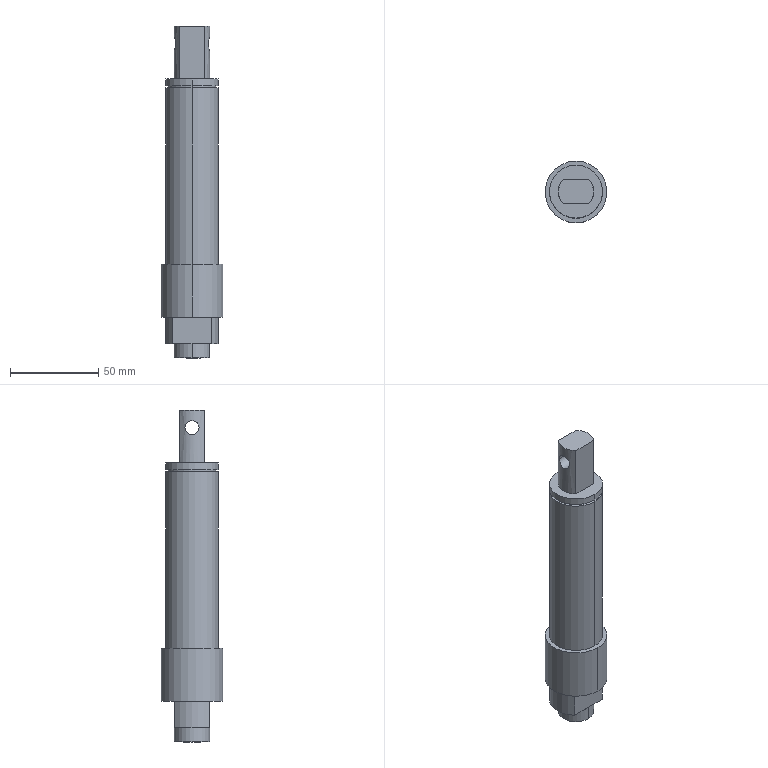Component | SolidWorks | -DrivenPulleyShaft-1 | 1 solid | 33 faces | box 35 x 35 x 188 mm | volume 119550 mm3 | cylinder 18 | plane 13 | cone 2 | commonest cylinder face diameters 30 x6 20 x4 8 x2 6.8 x2 35 x2 27 x2
build123d program:
from build123d import *

# Parameters (mm, degrees)
SKETCH2_W             = 5.308
SKETCH2_H             = 29.965
SKETCH2_W_2           = 6.945
SKETCH2_H_2           = 31.552
CUT_EXTRUDE1_DEPTH    = 15
M8_TAPPED_HOLE1_D     = 6.8
M8_TAPPED_HOLE1_DEPTH = 22.25
M8_TAPPED_HOLE1_TIP   = 2.043
SKETCH5_W             = 20.068
SKETCH5_H             = 42.894
SKETCH5_W_2           = 13.481
SKETCH5_H_2           = 39.37
CUT_EXTRUDE3_DEPTH    = 30
M8_TAPPED_HOLE2_D     = 8


with BuildPart() as part:
    # Sketch1 → Revolve1 (revolve)
    with BuildSketch(Plane(origin=(0, 0, 0), x_dir=(1, 0, 0), z_dir=(0, 1, 0)), mode=Mode.PRIVATE) as revolve1_sk:
        Polygon((0, 0), (0, 10), (30, 10), (30, 15), (33.8, 15), (33.8, 13.5), (35, 13.5), (35, 15), (135, 15), (135, 17.5), (165, 17.5), (165, 15), (180, 15), (180, 10), (188, 10), (188, 0), align=None)
    revolve(revolve1_sk.sketch.rotate(Axis((-511.379, 0, 0), (1, 0, 0)), 180), axis=Axis((-511.379, 0, 0), (1, 0, 0)))

    # Sketch2 → Cut-Extrude1 (cut)
    with BuildSketch(Plane(origin=(180, 0, 0), x_dir=(0, 0, -1), z_dir=(1, 0, 0))):
        with Locations((-12.654, -0.3473)):
            Rectangle(SKETCH2_W, SKETCH2_H)
        with Locations((13.473, -1.141)):
            Rectangle(SKETCH2_W_2, SKETCH2_H_2)
    extrude(amount=-CUT_EXTRUDE1_DEPTH, mode=Mode.SUBTRACT)

    # M8 Tapped Hole1
    with Locations(Plane(origin=(188, 0, 0), x_dir=(0, 0, -1), z_dir=(1, 0, 0))):
        with Locations((0, 0)):
            Hole(M8_TAPPED_HOLE1_D / 2, depth=M8_TAPPED_HOLE1_DEPTH)
            with Locations((0, 0, -(M8_TAPPED_HOLE1_DEPTH + M8_TAPPED_HOLE1_TIP / 2))):  # 118° drill point
                Cone(0, M8_TAPPED_HOLE1_D / 2, M8_TAPPED_HOLE1_TIP, mode=Mode.SUBTRACT)

    # Sketch5 → Cut-Extrude3 (cut)
    with BuildSketch(Plane.ZY):
        with Locations((-17.034, -1.358)):
            Rectangle(SKETCH5_W, SKETCH5_H)
        with Locations((13.74, -4.805)):
            Rectangle(SKETCH5_W_2, SKETCH5_H_2)
    extrude(amount=-CUT_EXTRUDE3_DEPTH, mode=Mode.SUBTRACT)

    # M8 Tapped Hole2 (through all)
    with Locations(Plane(origin=(0, -10, 0), x_dir=(-1, 0, 0), z_dir=(0, -1, 0))):
        with Locations((-10, 0)):
            Hole(M8_TAPPED_HOLE2_D / 2)


solid = part.part

# Placed as in the assembly
solid = solid.moved(Location((-130, 1094.5, 170), (90, 0, -90)))
STEP:
#1=COLOUR_RGB('',0.7922,0.8196,0.9333);
#2=FILL_AREA_STYLE_COLOUR('',#1);
#3=FILL_AREA_STYLE('',(#2));
#4=SURFACE_STYLE_FILL_AREA(#3);
#5=SURFACE_SIDE_STYLE('',(#4));
#6=SURFACE_STYLE_USAGE(.BOTH.,#5);
#7=PRESENTATION_STYLE_ASSIGNMENT((#6));
#8=CARTESIAN_POINT('',(-5.479,43.248,6.299));
#9=VERTEX_POINT('',#8);
#10=CARTESIAN_POINT('',(-5.479,42.933,6.299));
#11=VERTEX_POINT('',#10);
#12=CARTESIAN_POINT('',(-5.479,43.248,6.299));
#13=CARTESIAN_POINT('',(-5.479,43.248,6.31));
#14=CARTESIAN_POINT('',(-5.479,43.247,6.32));
#15=CARTESIAN_POINT('',(-5.481,43.243,6.34));
#16=CARTESIAN_POINT('',(-5.482,43.24,6.35));
#17=CARTESIAN_POINT('',(-5.486,43.232,6.369));
#18=CARTESIAN_POINT('',(-5.487,43.227,6.378));
#19=CARTESIAN_POINT('',(-5.491,43.216,6.395));
#20=CARTESIAN_POINT('',(-5.494,43.209,6.403));
#21=CARTESIAN_POINT('',(-5.498,43.195,6.418));
#22=CARTESIAN_POINT('',(-5.5,43.187,6.424));
#23=CARTESIAN_POINT('',(-5.504,43.17,6.436));
#24=CARTESIAN_POINT('',(-5.506,43.161,6.441));
#25=CARTESIAN_POINT('',(-5.509,43.142,6.449));
#26=CARTESIAN_POINT('',(-5.51,43.132,6.452));
#27=CARTESIAN_POINT('',(-5.511,43.112,6.456));
#28=CARTESIAN_POINT('',(-5.512,43.101,6.457));
#29=CARTESIAN_POINT('',(-5.512,43.08,6.457));
#30=CARTESIAN_POINT('',(-5.511,43.07,6.456));
#31=CARTESIAN_POINT('',(-5.51,43.049,6.452));
#32=CARTESIAN_POINT('',(-5.509,43.039,6.449));
#33=CARTESIAN_POINT('',(-5.506,43.021,6.441));
#34=CARTESIAN_POINT('',(-5.504,43.011,6.436));
#35=CARTESIAN_POINT('',(-5.5,42.994,6.424));
#36=CARTESIAN_POINT('',(-5.498,42.986,6.418));
#37=CARTESIAN_POINT('',(-5.494,42.972,6.403));
#38=CARTESIAN_POINT('',(-5.491,42.965,6.395));
#39=CARTESIAN_POINT('',(-5.487,42.954,6.379));
#40=CARTESIAN_POINT('',(-5.486,42.949,6.37));
#41=CARTESIAN_POINT('',(-5.482,42.941,6.35));
#42=CARTESIAN_POINT('',(-5.481,42.938,6.34));
#43=CARTESIAN_POINT('',(-5.479,42.934,6.32));
#44=CARTESIAN_POINT('',(-5.479,42.933,6.31));
#45=CARTESIAN_POINT('',(-5.479,42.933,6.299));
#46=B_SPLINE_CURVE_WITH_KNOTS('',3,(#12,#13,#14,#15,#16,#17,#18,#19,#20,#21,#22,#23,#24,#25,#26,#27,#28,#29,#30,#31,#32,#33,#34,#35,#36,#37,#38,#39,#40,#41,#42,#43,#44,#45),.UNSPECIFIED.,.F.,.F.,(4,2,2,2,2,2,2,2,2,2,2,2,2,2,2,2,4),(0.01264,0.01343,0.01422,0.01501,0.0158,0.01658,0.01737,0.01816,0.01895,0.01974,0.02053,0.02132,0.02211,0.0229,0.02369,0.02448,0.02527),.UNSPECIFIED.);
#47=EDGE_CURVE('',#9,#11,#46,.T.);
#48=ORIENTED_EDGE('',*,*,#47,.F.);
#49=CARTESIAN_POINT('',(-4.757,43.248,6.299));
#50=VERTEX_POINT('',#49);
#51=CARTESIAN_POINT('',(-4.724,43.248,6.299));
#52=DIRECTION('',(1.,0.,-0.));
#53=VECTOR('',#52,39.37);
#54=LINE('',#51,#53);
#55=EDGE_CURVE('',#9,#50,#54,.T.);
#56=ORIENTED_EDGE('',*,*,#55,.T.);
#57=CARTESIAN_POINT('',(-4.757,42.933,6.299));
#58=VERTEX_POINT('',#57);
#59=CARTESIAN_POINT('',(-4.757,42.933,6.299));
#60=CARTESIAN_POINT('',(-4.757,42.933,6.31));
#61=CARTESIAN_POINT('',(-4.757,42.934,6.32));
#62=CARTESIAN_POINT('',(-4.755,42.938,6.34));
#63=CARTESIAN_POINT('',(-4.754,42.941,6.35));
#64=CARTESIAN_POINT('',(-4.751,42.949,6.369));
#65=CARTESIAN_POINT('',(-4.749,42.954,6.378));
#66=CARTESIAN_POINT('',(-4.745,42.965,6.395));
#67=CARTESIAN_POINT('',(-4.743,42.972,6.403));
#68=CARTESIAN_POINT('',(-4.738,42.986,6.418));
#69=CARTESIAN_POINT('',(-4.736,42.994,6.424));
#70=CARTESIAN_POINT('',(-4.732,43.011,6.436));
#71=CARTESIAN_POINT('',(-4.731,43.02,6.441));
#72=CARTESIAN_POINT('',(-4.728,43.039,6.448));
#73=CARTESIAN_POINT('',(-4.726,43.049,6.452));
#74=CARTESIAN_POINT('',(-4.725,43.07,6.456));
#75=CARTESIAN_POINT('',(-4.724,43.08,6.457));
#76=CARTESIAN_POINT('',(-4.724,43.101,6.457));
#77=CARTESIAN_POINT('',(-4.725,43.111,6.456));
#78=CARTESIAN_POINT('',(-4.726,43.132,6.452));
#79=CARTESIAN_POINT('',(-4.728,43.142,6.449));
#80=CARTESIAN_POINT('',(-4.731,43.161,6.441));
#81=CARTESIAN_POINT('',(-4.732,43.17,6.436));
#82=CARTESIAN_POINT('',(-4.736,43.187,6.424));
#83=CARTESIAN_POINT('',(-4.738,43.195,6.418));
#84=CARTESIAN_POINT('',(-4.743,43.209,6.403));
#85=CARTESIAN_POINT('',(-4.745,43.216,6.395));
#86=CARTESIAN_POINT('',(-4.749,43.227,6.378));
#87=CARTESIAN_POINT('',(-4.751,43.232,6.369));
#88=CARTESIAN_POINT('',(-4.754,43.24,6.35));
#89=CARTESIAN_POINT('',(-4.755,43.243,6.34));
#90=CARTESIAN_POINT('',(-4.757,43.247,6.32));
#91=CARTESIAN_POINT('',(-4.757,43.248,6.31));
#92=CARTESIAN_POINT('',(-4.757,43.248,6.299));
#93=B_SPLINE_CURVE_WITH_KNOTS('',3,(#59,#60,#61,#62,#63,#64,#65,#66,#67,#68,#69,#70,#71,#72,#73,#74,#75,#76,#77,#78,#79,#80,#81,#82,#83,#84,#85,#86,#87,#88,#89,#90,#91,#92),.UNSPECIFIED.,.F.,.F.,(4,2,2,2,2,2,2,2,2,2,2,2,2,2,2,2,4),(0.,0.0007899,0.00158,0.00237,0.00316,0.00395,0.00474,0.00553,0.006319,0.007109,0.007899,0.008689,0.009479,0.01027,0.01106,0.01185,0.01264),.UNSPECIFIED.);
#94=EDGE_CURVE('',#58,#50,#93,.T.);
#95=ORIENTED_EDGE('',*,*,#94,.F.);
#96=CARTESIAN_POINT('',(-4.724,42.933,6.299));
#97=DIRECTION('',(1.,0.,-0.));
#98=VECTOR('',#97,39.37);
#99=LINE('',#96,#98);
#100=EDGE_CURVE('',#11,#58,#99,.T.);
#101=ORIENTED_EDGE('',*,*,#100,.F.);
#102=EDGE_LOOP('',(#48,#56,#95,#101));
#103=FACE_OUTER_BOUND('',#102,.T.);
#104=CARTESIAN_POINT('',(-4.724,43.091,6.299));
#105=DIRECTION('',(1.,0.,-0.));
#106=DIRECTION('',(0.,-1.,0.));
#107=AXIS2_PLACEMENT_3D('',#104,#105,#106);
#108=CYLINDRICAL_SURFACE('',#107,0.1575);
#109=ADVANCED_FACE('',(#103),#108,.F.);
#110=CARTESIAN_POINT('',(-5.118,43.224,0.1673));
#111=VERTEX_POINT('',#110);
#112=CARTESIAN_POINT('',(-5.118,42.957,0.1673));
#113=VERTEX_POINT('',#112);
#114=CARTESIAN_POINT('',(-5.118,43.091,0.1673));
#115=DIRECTION('',(-0.,-0.,-1.));
#116=DIRECTION('',(0.,-1.,0.));
#117=AXIS2_PLACEMENT_3D('',#114,#115,#116);
#118=CIRCLE('',#117,0.1339);
#119=EDGE_CURVE('',#111,#113,#118,.T.);
#120=ORIENTED_EDGE('',*,*,#119,.F.);
#121=CARTESIAN_POINT('',(-5.118,43.224,-0.7087));
#122=VERTEX_POINT('',#121);
#123=CARTESIAN_POINT('',(-5.118,43.224,-0.7087));
#124=DIRECTION('',(-0.,-0.,-1.));
#125=VECTOR('',#124,39.37);
#126=LINE('',#123,#125);
#127=EDGE_CURVE('',#111,#122,#126,.T.);
#128=ORIENTED_EDGE('',*,*,#127,.T.);
#129=CARTESIAN_POINT('',(-5.118,42.957,-0.7087));
#130=VERTEX_POINT('',#129);
#131=CARTESIAN_POINT('',(-5.118,43.091,-0.7087));
#132=DIRECTION('',(-0.,-0.,-1.));
#133=DIRECTION('',(0.,-1.,0.));
#134=AXIS2_PLACEMENT_3D('',#131,#132,#133);
#135=CIRCLE('',#134,0.1339);
#136=EDGE_CURVE('',#122,#130,#135,.T.);
#137=ORIENTED_EDGE('',*,*,#136,.T.);
#138=CARTESIAN_POINT('',(-5.118,42.957,-0.7087));
#139=DIRECTION('',(-0.,-0.,-1.));
#140=VECTOR('',#139,39.37);
#141=LINE('',#138,#140);
#142=EDGE_CURVE('',#113,#130,#141,.T.);
#143=ORIENTED_EDGE('',*,*,#142,.F.);
#144=EDGE_LOOP('',(#120,#128,#137,#143));
#145=FACE_OUTER_BOUND('',#144,.T.);
#146=CARTESIAN_POINT('',(-5.118,43.091,-0.7087));
#147=DIRECTION('',(-0.,-0.,-1.));
#148=DIRECTION('',(0.,-1.,0.));
#149=AXIS2_PLACEMENT_3D('',#146,#147,#148);
#150=CYLINDRICAL_SURFACE('',#149,0.1339);
#151=ADVANCED_FACE('',(#145),#150,.F.);
#152=CARTESIAN_POINT('',(-5.118,43.091,0.2478));
#153=VERTEX_POINT('',#152);
#154=CARTESIAN_POINT('',(-5.118,42.957,0.1673));
#155=DIRECTION('',(0.,-0.8572,-0.515));
#156=VECTOR('',#155,39.37);
#157=LINE('',#154,#156);
#158=EDGE_CURVE('',#153,#113,#157,.T.);
#159=ORIENTED_EDGE('',*,*,#158,.F.);
#160=CARTESIAN_POINT('',(-5.118,43.224,0.1673));
#161=DIRECTION('',(-0.,0.8572,-0.515));
#162=VECTOR('',#161,39.37);
#163=LINE('',#160,#162);
#164=EDGE_CURVE('',#153,#111,#163,.T.);
#165=ORIENTED_EDGE('',*,*,#164,.T.);
#166=ORIENTED_EDGE('',*,*,#119,.T.);
#167=EDGE_LOOP('',(#159,#165,#166));
#168=FACE_OUTER_BOUND('',#167,.T.);
#169=CARTESIAN_POINT('',(-5.118,43.091,0.1673));
#170=DIRECTION('',(-0.,-0.,-1.));
#171=DIRECTION('',(0.,-1.,0.));
#172=AXIS2_PLACEMENT_3D('',#169,#170,#171);
#173=CONICAL_SURFACE('',#172,0.1339,1.03);
#174=ADVANCED_FACE('',(#168),#173,.F.);
#175=CARTESIAN_POINT('',(-5.118,43.484,-0.7087));
#176=VERTEX_POINT('',#175);
#177=CARTESIAN_POINT('',(-5.118,42.697,-0.7087));
#178=VERTEX_POINT('',#177);
#179=CARTESIAN_POINT('',(-5.118,43.091,-0.7087));
#180=DIRECTION('',(0.,0.,1.));
#181=DIRECTION('',(-0.,1.,0.));
#182=AXIS2_PLACEMENT_3D('',#179,#180,#181);
#183=CIRCLE('',#182,0.3937);
#184=EDGE_CURVE('',#176,#178,#183,.T.);
#185=ORIENTED_EDGE('',*,*,#184,.T.);
#186=CARTESIAN_POINT('',(-5.118,42.697,-0.3937));
#187=VERTEX_POINT('',#186);
#188=CARTESIAN_POINT('',(-5.118,42.697,26.826));
#189=DIRECTION('',(0.,0.,1.));
#190=VECTOR('',#189,39.37);
#191=LINE('',#188,#190);
#192=EDGE_CURVE('',#178,#187,#191,.T.);
#193=ORIENTED_EDGE('',*,*,#192,.T.);
#194=CARTESIAN_POINT('',(-5.118,43.484,-0.3937));
#195=VERTEX_POINT('',#194);
#196=CARTESIAN_POINT('',(-5.118,43.091,-0.3937));
#197=DIRECTION('',(0.,0.,1.));
#198=DIRECTION('',(-0.,1.,0.));
#199=AXIS2_PLACEMENT_3D('',#196,#197,#198);
#200=CIRCLE('',#199,0.3937);
#201=EDGE_CURVE('',#195,#187,#200,.T.);
#202=ORIENTED_EDGE('',*,*,#201,.F.);
#203=CARTESIAN_POINT('',(-5.118,43.484,26.826));
#204=DIRECTION('',(0.,0.,1.));
#205=VECTOR('',#204,39.37);
#206=LINE('',#203,#205);
#207=EDGE_CURVE('',#176,#195,#206,.T.);
#208=ORIENTED_EDGE('',*,*,#207,.F.);
#209=EDGE_LOOP('',(#185,#193,#202,#208));
#210=FACE_OUTER_BOUND('',#209,.T.);
#211=CARTESIAN_POINT('',(-5.118,43.091,26.826));
#212=DIRECTION('',(0.,0.,1.));
#213=DIRECTION('',(-0.,1.,0.));
#214=AXIS2_PLACEMENT_3D('',#211,#212,#213);
#215=CYLINDRICAL_SURFACE('',#214,0.3937);
#216=ADVANCED_FACE('',(#210),#215,.T.);
#217=CARTESIAN_POINT('',(-5.118,43.78,0.1969));
#218=VERTEX_POINT('',#217);
#219=CARTESIAN_POINT('',(-5.118,42.402,0.1969));
#220=VERTEX_POINT('',#219);
#221=CARTESIAN_POINT('',(-5.118,43.091,0.1969));
#222=DIRECTION('',(0.,0.,1.));
#223=DIRECTION('',(-0.,1.,0.));
#224=AXIS2_PLACEMENT_3D('',#221,#222,#223);
#225=CIRCLE('',#224,0.689);
#226=EDGE_CURVE('',#218,#220,#225,.T.);
#227=ORIENTED_EDGE('',*,*,#226,.T.);
#228=CARTESIAN_POINT('',(-5.118,42.402,1.378));
#229=VERTEX_POINT('',#228);
#230=CARTESIAN_POINT('',(-5.118,42.402,26.826));
#231=DIRECTION('',(0.,0.,1.));
#232=VECTOR('',#231,39.37);
#233=LINE('',#230,#232);
#234=EDGE_CURVE('',#220,#229,#233,.T.);
#235=ORIENTED_EDGE('',*,*,#234,.T.);
#236=CARTESIAN_POINT('',(-5.118,43.78,1.378));
#237=VERTEX_POINT('',#236);
#238=CARTESIAN_POINT('',(-5.118,43.091,1.378));
#239=DIRECTION('',(0.,0.,1.));
#240=DIRECTION('',(-0.,1.,0.));
#241=AXIS2_PLACEMENT_3D('',#238,#239,#240);
#242=CIRCLE('',#241,0.689);
#243=EDGE_CURVE('',#237,#229,#242,.T.);
#244=ORIENTED_EDGE('',*,*,#243,.F.);
#245=CARTESIAN_POINT('',(-5.118,43.78,26.826));
#246=DIRECTION('',(0.,0.,1.));
#247=VECTOR('',#246,39.37);
#248=LINE('',#245,#247);
#249=EDGE_CURVE('',#218,#237,#248,.T.);
#250=ORIENTED_EDGE('',*,*,#249,.F.);
#251=EDGE_LOOP('',(#227,#235,#244,#250));
#252=FACE_OUTER_BOUND('',#251,.T.);
#253=CARTESIAN_POINT('',(-5.118,43.091,26.826));
#254=DIRECTION('',(0.,0.,1.));
#255=DIRECTION('',(-0.,1.,0.));
#256=AXIS2_PLACEMENT_3D('',#253,#254,#255);
#257=CYLINDRICAL_SURFACE('',#256,0.689);
#258=ADVANCED_FACE('',(#252),#257,.T.);
#259=CARTESIAN_POINT('',(-5.118,43.681,1.378));
#260=VERTEX_POINT('',#259);
#261=CARTESIAN_POINT('',(-5.118,42.5,1.378));
#262=VERTEX_POINT('',#261);
#263=CARTESIAN_POINT('',(-5.118,43.091,1.378));
#264=DIRECTION('',(0.,0.,1.));
#265=DIRECTION('',(-0.,1.,0.));
#266=AXIS2_PLACEMENT_3D('',#263,#264,#265);
#267=CIRCLE('',#266,0.5906);
#268=EDGE_CURVE('',#260,#262,#267,.T.);
#269=ORIENTED_EDGE('',*,*,#268,.T.);
#270=CARTESIAN_POINT('',(-5.118,42.5,5.315));
#271=VERTEX_POINT('',#270);
#272=CARTESIAN_POINT('',(-5.118,42.5,26.826));
#273=DIRECTION('',(0.,0.,1.));
#274=VECTOR('',#273,39.37);
#275=LINE('',#272,#274);
#276=EDGE_CURVE('',#262,#271,#275,.T.);
#277=ORIENTED_EDGE('',*,*,#276,.T.);
#278=CARTESIAN_POINT('',(-5.118,43.681,5.315));
#279=VERTEX_POINT('',#278);
#280=CARTESIAN_POINT('',(-5.118,43.091,5.315));
#281=DIRECTION('',(0.,0.,1.));
#282=DIRECTION('',(-0.,1.,0.));
#283=AXIS2_PLACEMENT_3D('',#280,#281,#282);
#284=CIRCLE('',#283,0.5906);
#285=EDGE_CURVE('',#279,#271,#284,.T.);
#286=ORIENTED_EDGE('',*,*,#285,.F.);
#287=CARTESIAN_POINT('',(-5.118,43.681,26.826));
#288=DIRECTION('',(0.,0.,1.));
#289=VECTOR('',#288,39.37);
#290=LINE('',#287,#289);
#291=EDGE_CURVE('',#260,#279,#290,.T.);
#292=ORIENTED_EDGE('',*,*,#291,.F.);
#293=EDGE_LOOP('',(#269,#277,#286,#292));
#294=FACE_OUTER_BOUND('',#293,.T.);
#295=CARTESIAN_POINT('',(-5.118,43.091,26.826));
#296=DIRECTION('',(0.,0.,1.));
#297=DIRECTION('',(-0.,1.,0.));
#298=AXIS2_PLACEMENT_3D('',#295,#296,#297);
#299=CYLINDRICAL_SURFACE('',#298,0.5906);
#300=ADVANCED_FACE('',(#294),#299,.T.);
#301=CARTESIAN_POINT('',(-5.118,43.622,5.315));
#302=VERTEX_POINT('',#301);
#303=CARTESIAN_POINT('',(-5.118,42.559,5.315));
#304=VERTEX_POINT('',#303);
#305=CARTESIAN_POINT('',(-5.118,43.091,5.315));
#306=DIRECTION('',(0.,0.,1.));
#307=DIRECTION('',(-0.,1.,0.));
#308=AXIS2_PLACEMENT_3D('',#305,#306,#307);
#309=CIRCLE('',#308,0.5315);
#310=EDGE_CURVE('',#302,#304,#309,.T.);
#311=ORIENTED_EDGE('',*,*,#310,.T.);
#312=CARTESIAN_POINT('',(-5.118,42.559,5.362));
#313=VERTEX_POINT('',#312);
#314=CARTESIAN_POINT('',(-5.118,42.559,26.826));
#315=DIRECTION('',(0.,0.,1.));
#316=VECTOR('',#315,39.37);
#317=LINE('',#314,#316);
#318=EDGE_CURVE('',#304,#313,#317,.T.);
#319=ORIENTED_EDGE('',*,*,#318,.T.);
#320=CARTESIAN_POINT('',(-5.118,43.622,5.362));
#321=VERTEX_POINT('',#320);
#322=CARTESIAN_POINT('',(-5.118,43.091,5.362));
#323=DIRECTION('',(0.,0.,1.));
#324=DIRECTION('',(-0.,1.,0.));
#325=AXIS2_PLACEMENT_3D('',#322,#323,#324);
#326=CIRCLE('',#325,0.5315);
#327=EDGE_CURVE('',#321,#313,#326,.T.);
#328=ORIENTED_EDGE('',*,*,#327,.F.);
#329=CARTESIAN_POINT('',(-5.118,43.622,26.826));
#330=DIRECTION('',(0.,0.,1.));
#331=VECTOR('',#330,39.37);
#332=LINE('',#329,#331);
#333=EDGE_CURVE('',#302,#321,#332,.T.);
#334=ORIENTED_EDGE('',*,*,#333,.F.);
#335=EDGE_LOOP('',(#311,#319,#328,#334));
#336=FACE_OUTER_BOUND('',#335,.T.);
#337=CARTESIAN_POINT('',(-5.118,43.091,26.826));
#338=DIRECTION('',(0.,0.,1.));
#339=DIRECTION('',(-0.,1.,0.));
#340=AXIS2_PLACEMENT_3D('',#337,#338,#339);
#341=CYLINDRICAL_SURFACE('',#340,0.5315);
#342=ADVANCED_FACE('',(#336),#341,.T.);
#343=CARTESIAN_POINT('',(-5.118,43.681,5.362));
#344=VERTEX_POINT('',#343);
#345=CARTESIAN_POINT('',(-5.118,42.5,5.362));
#346=VERTEX_POINT('',#345);
#347=CARTESIAN_POINT('',(-5.118,43.091,5.362));
#348=DIRECTION('',(0.,0.,1.));
#349=DIRECTION('',(-0.,1.,0.));
#350=AXIS2_PLACEMENT_3D('',#347,#348,#349);
#351=CIRCLE('',#350,0.5906);
#352=EDGE_CURVE('',#344,#346,#351,.T.);
#353=ORIENTED_EDGE('',*,*,#352,.T.);
#354=CARTESIAN_POINT('',(-5.118,42.5,5.512));
#355=VERTEX_POINT('',#354);
#356=CARTESIAN_POINT('',(-5.118,42.5,26.826));
#357=DIRECTION('',(0.,0.,1.));
#358=VECTOR('',#357,39.37);
#359=LINE('',#356,#358);
#360=EDGE_CURVE('',#346,#355,#359,.T.);
#361=ORIENTED_EDGE('',*,*,#360,.T.);
#362=CARTESIAN_POINT('',(-5.118,43.681,5.512));
#363=VERTEX_POINT('',#362);
#364=CARTESIAN_POINT('',(-5.118,43.091,5.512));
#365=DIRECTION('',(0.,0.,1.));
#366=DIRECTION('',(-0.,1.,0.));
#367=AXIS2_PLACEMENT_3D('',#364,#365,#366);
#368=CIRCLE('',#367,0.5906);
#369=EDGE_CURVE('',#363,#355,#368,.T.);
#370=ORIENTED_EDGE('',*,*,#369,.F.);
#371=CARTESIAN_POINT('',(-5.118,43.681,26.826));
#372=DIRECTION('',(0.,0.,1.));
#373=VECTOR('',#372,39.37);
#374=LINE('',#371,#373);
#375=EDGE_CURVE('',#344,#363,#374,.T.);
#376=ORIENTED_EDGE('',*,*,#375,.F.);
#377=EDGE_LOOP('',(#353,#361,#370,#376));
#378=FACE_OUTER_BOUND('',#377,.T.);
#379=CARTESIAN_POINT('',(-5.118,43.091,26.826));
#380=DIRECTION('',(0.,0.,1.));
#381=DIRECTION('',(-0.,1.,0.));
#382=AXIS2_PLACEMENT_3D('',#379,#380,#381);
#383=CYLINDRICAL_SURFACE('',#382,0.5906);
#384=ADVANCED_FACE('',(#378),#383,.T.);
#385=ORIENTED_EDGE('',*,*,#94,.T.);
#386=CARTESIAN_POINT('',(-4.757,43.248,6.299));
#387=CARTESIAN_POINT('',(-4.757,43.248,6.289));
#388=CARTESIAN_POINT('',(-4.757,43.247,6.278));
#389=CARTESIAN_POINT('',(-4.755,43.243,6.258));
#390=CARTESIAN_POINT('',(-4.754,43.24,6.248));
#391=CARTESIAN_POINT('',(-4.751,43.232,6.229));
#392=CARTESIAN_POINT('',(-4.749,43.227,6.22));
#393=CARTESIAN_POINT('',(-4.745,43.216,6.203));
#394=CARTESIAN_POINT('',(-4.743,43.209,6.195));
#395=CARTESIAN_POINT('',(-4.738,43.195,6.181));
#396=CARTESIAN_POINT('',(-4.736,43.187,6.174));
#397=CARTESIAN_POINT('',(-4.732,43.17,6.163));
#398=CARTESIAN_POINT('',(-4.731,43.161,6.158));
#399=CARTESIAN_POINT('',(-4.728,43.142,6.15));
#400=CARTESIAN_POINT('',(-4.726,43.132,6.147));
#401=CARTESIAN_POINT('',(-4.725,43.112,6.143));
#402=CARTESIAN_POINT('',(-4.724,43.101,6.142));
#403=CARTESIAN_POINT('',(-4.724,43.08,6.142));
#404=CARTESIAN_POINT('',(-4.725,43.07,6.143));
#405=CARTESIAN_POINT('',(-4.726,43.049,6.147));
#406=CARTESIAN_POINT('',(-4.728,43.039,6.15));
#407=CARTESIAN_POINT('',(-4.731,43.021,6.158));
#408=CARTESIAN_POINT('',(-4.732,43.011,6.163));
#409=CARTESIAN_POINT('',(-4.736,42.994,6.174));
#410=CARTESIAN_POINT('',(-4.738,42.986,6.181));
#411=CARTESIAN_POINT('',(-4.743,42.972,6.195));
#412=CARTESIAN_POINT('',(-4.745,42.965,6.203));
#413=CARTESIAN_POINT('',(-4.749,42.954,6.22));
#414=CARTESIAN_POINT('',(-4.751,42.949,6.229));
#415=CARTESIAN_POINT('',(-4.754,42.941,6.248));
#416=CARTESIAN_POINT('',(-4.755,42.938,6.258));
#417=CARTESIAN_POINT('',(-4.757,42.934,6.278));
#418=CARTESIAN_POINT('',(-4.757,42.933,6.289));
#419=CARTESIAN_POINT('',(-4.757,42.933,6.299));
#420=B_SPLINE_CURVE_WITH_KNOTS('',3,(#386,#387,#388,#389,#390,#391,#392,#393,#394,#395,#396,#397,#398,#399,#400,#401,#402,#403,#404,#405,#406,#407,#408,#409,#410,#411,#412,#413,#414,#415,#416,#417,#418,#419),.UNSPECIFIED.,.F.,.F.,(4,2,2,2,2,2,2,2,2,2,2,2,2,2,2,2,4),(0.01264,0.01343,0.01422,0.01501,0.0158,0.01658,0.01737,0.01816,0.01895,0.01974,0.02053,0.02132,0.02211,0.0229,0.02369,0.02448,0.02527),.UNSPECIFIED.);
#421=EDGE_CURVE('',#50,#58,#420,.T.);
#422=ORIENTED_EDGE('',*,*,#421,.T.);
#423=EDGE_LOOP('',(#385,#422));
#424=FACE_BOUND('',#423,.T.);
#425=CARTESIAN_POINT('',(-4.837,42.815,5.512));
#426=VERTEX_POINT('',#425);
#427=CARTESIAN_POINT('',(-4.837,43.366,5.512));
#428=VERTEX_POINT('',#427);
#429=CARTESIAN_POINT('',(-5.118,43.091,5.512));
#430=DIRECTION('',(0.,0.,1.));
#431=DIRECTION('',(-0.,1.,0.));
#432=AXIS2_PLACEMENT_3D('',#429,#430,#431);
#433=CIRCLE('',#432,0.3937);
#434=EDGE_CURVE('',#426,#428,#433,.T.);
#435=ORIENTED_EDGE('',*,*,#434,.T.);
#436=CARTESIAN_POINT('',(-4.837,43.366,6.693));
#437=VERTEX_POINT('',#436);
#438=CARTESIAN_POINT('',(-4.837,43.366,26.826));
#439=DIRECTION('',(0.,0.,1.));
#440=VECTOR('',#439,39.37);
#441=LINE('',#438,#440);
#442=EDGE_CURVE('',#428,#437,#441,.T.);
#443=ORIENTED_EDGE('',*,*,#442,.T.);
#444=CARTESIAN_POINT('',(-4.837,42.815,6.693));
#445=VERTEX_POINT('',#444);
#446=CARTESIAN_POINT('',(-5.118,43.091,6.693));
#447=DIRECTION('',(0.,0.,1.));
#448=DIRECTION('',(-0.,1.,0.));
#449=AXIS2_PLACEMENT_3D('',#446,#447,#448);
#450=CIRCLE('',#449,0.3937);
#451=EDGE_CURVE('',#445,#437,#450,.T.);
#452=ORIENTED_EDGE('',*,*,#451,.F.);
#453=CARTESIAN_POINT('',(-4.837,42.815,26.826));
#454=DIRECTION('',(-0.,-0.,-1.));
#455=VECTOR('',#454,39.37);
#456=LINE('',#453,#455);
#457=EDGE_CURVE('',#445,#426,#456,.T.);
#458=ORIENTED_EDGE('',*,*,#457,.T.);
#459=EDGE_LOOP('',(#435,#443,#452,#458));
#460=FACE_OUTER_BOUND('',#459,.T.);
#461=CARTESIAN_POINT('',(-5.118,43.091,26.826));
#462=DIRECTION('',(0.,0.,1.));
#463=DIRECTION('',(-0.,1.,0.));
#464=AXIS2_PLACEMENT_3D('',#461,#462,#463);
#465=CYLINDRICAL_SURFACE('',#464,0.3937);
#466=ADVANCED_FACE('',(#424,#460),#465,.T.);
#467=CARTESIAN_POINT('',(-5.558,43.484,-0.3937));
#468=VERTEX_POINT('',#467);
#469=CARTESIAN_POINT('',(-5.558,42.697,-0.3937));
#470=VERTEX_POINT('',#469);
#471=CARTESIAN_POINT('',(-5.118,43.091,-0.3937));
#472=DIRECTION('',(0.,0.,1.));
#473=DIRECTION('',(-0.,1.,0.));
#474=AXIS2_PLACEMENT_3D('',#471,#472,#473);
#475=CIRCLE('',#474,0.5906);
#476=EDGE_CURVE('',#468,#470,#475,.T.);
#477=ORIENTED_EDGE('',*,*,#476,.T.);
#478=CARTESIAN_POINT('',(-5.558,42.697,0.1969));
#479=VERTEX_POINT('',#478);
#480=CARTESIAN_POINT('',(-5.558,42.697,26.826));
#481=DIRECTION('',(0.,0.,1.));
#482=VECTOR('',#481,39.37);
#483=LINE('',#480,#482);
#484=EDGE_CURVE('',#470,#479,#483,.T.);
#485=ORIENTED_EDGE('',*,*,#484,.T.);
#486=CARTESIAN_POINT('',(-5.558,43.484,0.1969));
#487=VERTEX_POINT('',#486);
#488=CARTESIAN_POINT('',(-5.118,43.091,0.1969));
#489=DIRECTION('',(0.,0.,1.));
#490=DIRECTION('',(-0.,1.,0.));
#491=AXIS2_PLACEMENT_3D('',#488,#489,#490);
#492=CIRCLE('',#491,0.5906);
#493=EDGE_CURVE('',#487,#479,#492,.T.);
#494=ORIENTED_EDGE('',*,*,#493,.F.);
#495=CARTESIAN_POINT('',(-5.558,43.484,26.826));
#496=DIRECTION('',(-0.,-0.,-1.));
#497=VECTOR('',#496,39.37);
#498=LINE('',#495,#497);
#499=EDGE_CURVE('',#487,#468,#498,.T.);
#500=ORIENTED_EDGE('',*,*,#499,.T.);
#501=EDGE_LOOP('',(#477,#485,#494,#500));
#502=FACE_OUTER_BOUND('',#501,.T.);
#503=CARTESIAN_POINT('',(-5.118,43.091,26.826));
#504=DIRECTION('',(0.,0.,1.));
#505=DIRECTION('',(-0.,1.,0.));
#506=AXIS2_PLACEMENT_3D('',#503,#504,#505);
#507=CYLINDRICAL_SURFACE('',#506,0.5906);
#508=ADVANCED_FACE('',(#502),#507,.T.);
#509=CARTESIAN_POINT('',(-4.678,42.697,-0.3937));
#510=VERTEX_POINT('',#509);
#511=CARTESIAN_POINT('',(-4.678,43.484,-0.3937));
#512=VERTEX_POINT('',#511);
#513=CARTESIAN_POINT('',(-5.118,43.091,-0.3937));
#514=DIRECTION('',(0.,0.,1.));
#515=DIRECTION('',(-0.,1.,0.));
#516=AXIS2_PLACEMENT_3D('',#513,#514,#515);
#517=CIRCLE('',#516,0.5906);
#518=EDGE_CURVE('',#510,#512,#517,.T.);
#519=ORIENTED_EDGE('',*,*,#518,.F.);
#520=CARTESIAN_POINT('',(-5.694,42.697,-0.3937));
#521=DIRECTION('',(1.,0.,-0.));
#522=VECTOR('',#521,39.37);
#523=LINE('',#520,#522);
#524=EDGE_CURVE('',#187,#510,#523,.T.);
#525=ORIENTED_EDGE('',*,*,#524,.F.);
#526=CARTESIAN_POINT('',(-5.118,43.091,-0.3937));
#527=DIRECTION('',(0.,0.,1.));
#528=DIRECTION('',(-0.,1.,0.));
#529=AXIS2_PLACEMENT_3D('',#526,#527,#528);
#530=CIRCLE('',#529,0.3937);
#531=EDGE_CURVE('',#187,#195,#530,.T.);
#532=ORIENTED_EDGE('',*,*,#531,.T.);
#533=CARTESIAN_POINT('',(-5.694,43.484,-0.3937));
#534=DIRECTION('',(-1.,-0.,0.));
#535=VECTOR('',#534,39.37);
#536=LINE('',#533,#535);
#537=EDGE_CURVE('',#512,#195,#536,.T.);
#538=ORIENTED_EDGE('',*,*,#537,.F.);
#539=EDGE_LOOP('',(#519,#525,#532,#538));
#540=FACE_OUTER_BOUND('',#539,.T.);
#541=CARTESIAN_POINT('',(-5.118,42.5,-0.3937));
#542=DIRECTION('',(0.,0.,1.));
#543=DIRECTION('',(-0.,1.,-0.));
#544=AXIS2_PLACEMENT_3D('',#541,#542,#543);
#545=PLANE('',#544);
#546=ADVANCED_FACE('',(#540),#545,.F.);
#547=ORIENTED_EDGE('',*,*,#451,.T.);
#548=CARTESIAN_POINT('',(-5.399,43.366,6.693));
#549=VERTEX_POINT('',#548);
#550=CARTESIAN_POINT('',(-5.704,43.366,6.693));
#551=DIRECTION('',(1.,0.,-0.));
#552=VECTOR('',#551,39.37);
#553=LINE('',#550,#552);
#554=EDGE_CURVE('',#549,#437,#553,.T.);
#555=ORIENTED_EDGE('',*,*,#554,.F.);
#556=CARTESIAN_POINT('',(-5.399,42.815,6.693));
#557=VERTEX_POINT('',#556);
#558=CARTESIAN_POINT('',(-5.118,43.091,6.693));
#559=DIRECTION('',(0.,0.,1.));
#560=DIRECTION('',(-0.,1.,0.));
#561=AXIS2_PLACEMENT_3D('',#558,#559,#560);
#562=CIRCLE('',#561,0.3937);
#563=EDGE_CURVE('',#549,#557,#562,.T.);
#564=ORIENTED_EDGE('',*,*,#563,.T.);
#565=CARTESIAN_POINT('',(-5.909,42.815,6.693));
#566=DIRECTION('',(-1.,-0.,0.));
#567=VECTOR('',#566,39.37);
#568=LINE('',#565,#567);
#569=EDGE_CURVE('',#445,#557,#568,.T.);
#570=ORIENTED_EDGE('',*,*,#569,.F.);
#571=EDGE_LOOP('',(#547,#555,#564,#570));
#572=FACE_OUTER_BOUND('',#571,.T.);
#573=CARTESIAN_POINT('',(-5.118,43.091,6.693));
#574=DIRECTION('',(-0.,-0.,-1.));
#575=DIRECTION('',(0.,-1.,0.));
#576=AXIS2_PLACEMENT_3D('',#573,#574,#575);
#577=PLANE('',#576);
#578=ADVANCED_FACE('',(#572),#577,.F.);
#579=CARTESIAN_POINT('',(-5.479,42.933,6.299));
#580=CARTESIAN_POINT('',(-5.479,42.933,6.289));
#581=CARTESIAN_POINT('',(-5.479,42.934,6.278));
#582=CARTESIAN_POINT('',(-5.481,42.938,6.258));
#583=CARTESIAN_POINT('',(-5.482,42.941,6.248));
#584=CARTESIAN_POINT('',(-5.486,42.949,6.229));
#585=CARTESIAN_POINT('',(-5.487,42.954,6.22));
#586=CARTESIAN_POINT('',(-5.491,42.965,6.203));
#587=CARTESIAN_POINT('',(-5.494,42.972,6.195));
#588=CARTESIAN_POINT('',(-5.498,42.986,6.181));
#589=CARTESIAN_POINT('',(-5.5,42.994,6.174));
#590=CARTESIAN_POINT('',(-5.504,43.011,6.163));
#591=CARTESIAN_POINT('',(-5.506,43.02,6.158));
#592=CARTESIAN_POINT('',(-5.509,43.039,6.15));
#593=CARTESIAN_POINT('',(-5.51,43.049,6.147));
#594=CARTESIAN_POINT('',(-5.511,43.07,6.143));
#595=CARTESIAN_POINT('',(-5.512,43.08,6.142));
#596=CARTESIAN_POINT('',(-5.512,43.101,6.142));
#597=CARTESIAN_POINT('',(-5.511,43.111,6.143));
#598=CARTESIAN_POINT('',(-5.51,43.132,6.147));
#599=CARTESIAN_POINT('',(-5.509,43.142,6.15));
#600=CARTESIAN_POINT('',(-5.506,43.161,6.158));
#601=CARTESIAN_POINT('',(-5.504,43.17,6.163));
#602=CARTESIAN_POINT('',(-5.5,43.187,6.174));
#603=CARTESIAN_POINT('',(-5.498,43.195,6.181));
#604=CARTESIAN_POINT('',(-5.494,43.209,6.195));
#605=CARTESIAN_POINT('',(-5.491,43.216,6.203));
#606=CARTESIAN_POINT('',(-5.487,43.227,6.22));
#607=CARTESIAN_POINT('',(-5.486,43.232,6.229));
#608=CARTESIAN_POINT('',(-5.482,43.24,6.248));
#609=CARTESIAN_POINT('',(-5.481,43.243,6.258));
#610=CARTESIAN_POINT('',(-5.479,43.247,6.278));
#611=CARTESIAN_POINT('',(-5.479,43.248,6.289));
#612=CARTESIAN_POINT('',(-5.479,43.248,6.299));
#613=B_SPLINE_CURVE_WITH_KNOTS('',3,(#579,#580,#581,#582,#583,#584,#585,#586,#587,#588,#589,#590,#591,#592,#593,#594,#595,#596,#597,#598,#599,#600,#601,#602,#603,#604,#605,#606,#607,#608,#609,#610,#611,#612),.UNSPECIFIED.,.F.,.F.,(4,2,2,2,2,2,2,2,2,2,2,2,2,2,2,2,4),(0.,0.0007899,0.00158,0.00237,0.00316,0.00395,0.00474,0.00553,0.006319,0.007109,0.007899,0.008689,0.009479,0.01027,0.01106,0.01185,0.01264),.UNSPECIFIED.);
#614=EDGE_CURVE('',#11,#9,#613,.T.);
#615=ORIENTED_EDGE('',*,*,#614,.T.);
#616=ORIENTED_EDGE('',*,*,#47,.T.);
#617=EDGE_LOOP('',(#615,#616));
#618=FACE_BOUND('',#617,.T.);
#619=ORIENTED_EDGE('',*,*,#563,.F.);
#620=CARTESIAN_POINT('',(-5.399,43.366,5.512));
#621=VERTEX_POINT('',#620);
#622=CARTESIAN_POINT('',(-5.399,43.366,26.826));
#623=DIRECTION('',(-0.,-0.,-1.));
#624=VECTOR('',#623,39.37);
#625=LINE('',#622,#624);
#626=EDGE_CURVE('',#549,#621,#625,.T.);
#627=ORIENTED_EDGE('',*,*,#626,.T.);
#628=CARTESIAN_POINT('',(-5.399,42.815,5.512));
#629=VERTEX_POINT('',#628);
#630=CARTESIAN_POINT('',(-5.118,43.091,5.512));
#631=DIRECTION('',(0.,0.,1.));
#632=DIRECTION('',(-0.,1.,0.));
#633=AXIS2_PLACEMENT_3D('',#630,#631,#632);
#634=CIRCLE('',#633,0.3937);
#635=EDGE_CURVE('',#621,#629,#634,.T.);
#636=ORIENTED_EDGE('',*,*,#635,.T.);
#637=CARTESIAN_POINT('',(-5.399,42.815,26.826));
#638=DIRECTION('',(0.,0.,1.));
#639=VECTOR('',#638,39.37);
#640=LINE('',#637,#639);
#641=EDGE_CURVE('',#629,#557,#640,.T.);
#642=ORIENTED_EDGE('',*,*,#641,.T.);
#643=EDGE_LOOP('',(#619,#627,#636,#642));
#644=FACE_OUTER_BOUND('',#643,.T.);
#645=CARTESIAN_POINT('',(-5.118,43.091,26.826));
#646=DIRECTION('',(0.,0.,1.));
#647=DIRECTION('',(-0.,1.,0.));
#648=AXIS2_PLACEMENT_3D('',#645,#646,#647);
#649=CYLINDRICAL_SURFACE('',#648,0.3937);
#650=ADVANCED_FACE('',(#618,#644),#649,.T.);
#651=ORIENTED_EDGE('',*,*,#635,.F.);
#652=CARTESIAN_POINT('',(-5.704,43.366,5.512));
#653=DIRECTION('',(1.,0.,-0.));
#654=VECTOR('',#653,39.37);
#655=LINE('',#652,#654);
#656=EDGE_CURVE('',#621,#428,#655,.T.);
#657=ORIENTED_EDGE('',*,*,#656,.T.);
#658=ORIENTED_EDGE('',*,*,#434,.F.);
#659=CARTESIAN_POINT('',(-5.909,42.815,5.512));
#660=DIRECTION('',(-1.,-0.,0.));
#661=VECTOR('',#660,39.37);
#662=LINE('',#659,#661);
#663=EDGE_CURVE('',#426,#629,#662,.T.);
#664=ORIENTED_EDGE('',*,*,#663,.T.);
#665=EDGE_LOOP('',(#651,#657,#658,#664));
#666=FACE_BOUND('',#665,.T.);
#667=ORIENTED_EDGE('',*,*,#369,.T.);
#668=CARTESIAN_POINT('',(-5.118,43.091,5.512));
#669=DIRECTION('',(0.,0.,1.));
#670=DIRECTION('',(-0.,1.,0.));
#671=AXIS2_PLACEMENT_3D('',#668,#669,#670);
#672=CIRCLE('',#671,0.5906);
#673=EDGE_CURVE('',#355,#363,#672,.T.);
#674=ORIENTED_EDGE('',*,*,#673,.T.);
#675=EDGE_LOOP('',(#667,#674));
#676=FACE_OUTER_BOUND('',#675,.T.);
#677=CARTESIAN_POINT('',(-5.118,42.697,5.512));
#678=DIRECTION('',(-0.,-0.,-1.));
#679=DIRECTION('',(0.,-1.,0.));
#680=AXIS2_PLACEMENT_3D('',#677,#678,#679);
#681=PLANE('',#680);
#682=ADVANCED_FACE('',(#666,#676),#681,.F.);
#683=ORIENTED_EDGE('',*,*,#360,.F.);
#684=CARTESIAN_POINT('',(-5.118,43.091,5.362));
#685=DIRECTION('',(0.,0.,1.));
#686=DIRECTION('',(-0.,1.,0.));
#687=AXIS2_PLACEMENT_3D('',#684,#685,#686);
#688=CIRCLE('',#687,0.5906);
#689=EDGE_CURVE('',#346,#344,#688,.T.);
#690=ORIENTED_EDGE('',*,*,#689,.T.);
#691=ORIENTED_EDGE('',*,*,#375,.T.);
#692=ORIENTED_EDGE('',*,*,#673,.F.);
#693=EDGE_LOOP('',(#683,#690,#691,#692));
#694=FACE_OUTER_BOUND('',#693,.T.);
#695=CARTESIAN_POINT('',(-5.118,43.091,26.826));
#696=DIRECTION('',(0.,0.,1.));
#697=DIRECTION('',(-0.,1.,0.));
#698=AXIS2_PLACEMENT_3D('',#695,#696,#697);
#699=CYLINDRICAL_SURFACE('',#698,0.5906);
#700=ADVANCED_FACE('',(#694),#699,.T.);
#701=ORIENTED_EDGE('',*,*,#352,.F.);
#702=ORIENTED_EDGE('',*,*,#689,.F.);
#703=EDGE_LOOP('',(#701,#702));
#704=FACE_OUTER_BOUND('',#703,.T.);
#705=ORIENTED_EDGE('',*,*,#327,.T.);
#706=CARTESIAN_POINT('',(-5.118,43.091,5.362));
#707=DIRECTION('',(0.,0.,1.));
#708=DIRECTION('',(-0.,1.,0.));
#709=AXIS2_PLACEMENT_3D('',#706,#707,#708);
#710=CIRCLE('',#709,0.5315);
#711=EDGE_CURVE('',#313,#321,#710,.T.);
#712=ORIENTED_EDGE('',*,*,#711,.T.);
#713=EDGE_LOOP('',(#705,#712));
#714=FACE_BOUND('',#713,.T.);
#715=CARTESIAN_POINT('',(-5.118,42.5,5.362));
#716=DIRECTION('',(0.,0.,1.));
#717=DIRECTION('',(-0.,1.,-0.));
#718=AXIS2_PLACEMENT_3D('',#715,#716,#717);
#719=PLANE('',#718);
#720=ADVANCED_FACE('',(#704,#714),#719,.F.);
#721=ORIENTED_EDGE('',*,*,#318,.F.);
#722=CARTESIAN_POINT('',(-5.118,43.091,5.315));
#723=DIRECTION('',(0.,0.,1.));
#724=DIRECTION('',(-0.,1.,0.));
#725=AXIS2_PLACEMENT_3D('',#722,#723,#724);
#726=CIRCLE('',#725,0.5315);
#727=EDGE_CURVE('',#304,#302,#726,.T.);
#728=ORIENTED_EDGE('',*,*,#727,.T.);
#729=ORIENTED_EDGE('',*,*,#333,.T.);
#730=ORIENTED_EDGE('',*,*,#711,.F.);
#731=EDGE_LOOP('',(#721,#728,#729,#730));
#732=FACE_OUTER_BOUND('',#731,.T.);
#733=CARTESIAN_POINT('',(-5.118,43.091,26.826));
#734=DIRECTION('',(0.,0.,1.));
#735=DIRECTION('',(-0.,1.,0.));
#736=AXIS2_PLACEMENT_3D('',#733,#734,#735);
#737=CYLINDRICAL_SURFACE('',#736,0.5315);
#738=ADVANCED_FACE('',(#732),#737,.T.);
#739=ORIENTED_EDGE('',*,*,#310,.F.);
#740=ORIENTED_EDGE('',*,*,#727,.F.);
#741=EDGE_LOOP('',(#739,#740));
#742=FACE_BOUND('',#741,.T.);
#743=ORIENTED_EDGE('',*,*,#285,.T.);
#744=CARTESIAN_POINT('',(-5.118,43.091,5.315));
#745=DIRECTION('',(0.,0.,1.));
#746=DIRECTION('',(-0.,1.,0.));
#747=AXIS2_PLACEMENT_3D('',#744,#745,#746);
#748=CIRCLE('',#747,0.5906);
#749=EDGE_CURVE('',#271,#279,#748,.T.);
#750=ORIENTED_EDGE('',*,*,#749,.T.);
#751=EDGE_LOOP('',(#743,#750));
#752=FACE_OUTER_BOUND('',#751,.T.);
#753=CARTESIAN_POINT('',(-5.118,42.559,5.315));
#754=DIRECTION('',(-0.,-0.,-1.));
#755=DIRECTION('',(0.,-1.,0.));
#756=AXIS2_PLACEMENT_3D('',#753,#754,#755);
#757=PLANE('',#756);
#758=ADVANCED_FACE('',(#742,#752),#757,.F.);
#759=ORIENTED_EDGE('',*,*,#276,.F.);
#760=CARTESIAN_POINT('',(-5.118,43.091,1.378));
#761=DIRECTION('',(0.,0.,1.));
#762=DIRECTION('',(-0.,1.,0.));
#763=AXIS2_PLACEMENT_3D('',#760,#761,#762);
#764=CIRCLE('',#763,0.5906);
#765=EDGE_CURVE('',#262,#260,#764,.T.);
#766=ORIENTED_EDGE('',*,*,#765,.T.);
#767=ORIENTED_EDGE('',*,*,#291,.T.);
#768=ORIENTED_EDGE('',*,*,#749,.F.);
#769=EDGE_LOOP('',(#759,#766,#767,#768));
#770=FACE_OUTER_BOUND('',#769,.T.);
#771=CARTESIAN_POINT('',(-5.118,43.091,26.826));
#772=DIRECTION('',(0.,0.,1.));
#773=DIRECTION('',(-0.,1.,0.));
#774=AXIS2_PLACEMENT_3D('',#771,#772,#773);
#775=CYLINDRICAL_SURFACE('',#774,0.5906);
#776=ADVANCED_FACE('',(#770),#775,.T.);
#777=ORIENTED_EDGE('',*,*,#268,.F.);
#778=ORIENTED_EDGE('',*,*,#765,.F.);
#779=EDGE_LOOP('',(#777,#778));
#780=FACE_BOUND('',#779,.T.);
#781=ORIENTED_EDGE('',*,*,#243,.T.);
#782=CARTESIAN_POINT('',(-5.118,43.091,1.378));
#783=DIRECTION('',(0.,0.,1.));
#784=DIRECTION('',(-0.,1.,0.));
#785=AXIS2_PLACEMENT_3D('',#782,#783,#784);
#786=CIRCLE('',#785,0.689);
#787=EDGE_CURVE('',#229,#237,#786,.T.);
#788=ORIENTED_EDGE('',*,*,#787,.T.);
#789=EDGE_LOOP('',(#781,#788));
#790=FACE_OUTER_BOUND('',#789,.T.);
#791=CARTESIAN_POINT('',(-5.118,42.5,1.378));
#792=DIRECTION('',(-0.,-0.,-1.));
#793=DIRECTION('',(0.,-1.,0.));
#794=AXIS2_PLACEMENT_3D('',#791,#792,#793);
#795=PLANE('',#794);
#796=ADVANCED_FACE('',(#780,#790),#795,.F.);
#797=ORIENTED_EDGE('',*,*,#234,.F.);
#798=CARTESIAN_POINT('',(-5.118,43.091,0.1969));
#799=DIRECTION('',(0.,0.,1.));
#800=DIRECTION('',(-0.,1.,0.));
#801=AXIS2_PLACEMENT_3D('',#798,#799,#800);
#802=CIRCLE('',#801,0.689);
#803=EDGE_CURVE('',#220,#218,#802,.T.);
#804=ORIENTED_EDGE('',*,*,#803,.T.);
#805=ORIENTED_EDGE('',*,*,#249,.T.);
#806=ORIENTED_EDGE('',*,*,#787,.F.);
#807=EDGE_LOOP('',(#797,#804,#805,#806));
#808=FACE_OUTER_BOUND('',#807,.T.);
#809=CARTESIAN_POINT('',(-5.118,43.091,26.826));
#810=DIRECTION('',(0.,0.,1.));
#811=DIRECTION('',(-0.,1.,0.));
#812=AXIS2_PLACEMENT_3D('',#809,#810,#811);
#813=CYLINDRICAL_SURFACE('',#812,0.689);
#814=ADVANCED_FACE('',(#808),#813,.T.);
#815=CARTESIAN_POINT('',(-4.678,42.697,0.1969));
#816=VERTEX_POINT('',#815);
#817=CARTESIAN_POINT('',(-5.694,42.697,0.1969));
#818=DIRECTION('',(1.,0.,-0.));
#819=VECTOR('',#818,39.37);
#820=LINE('',#817,#819);
#821=EDGE_CURVE('',#479,#816,#820,.T.);
#822=ORIENTED_EDGE('',*,*,#821,.T.);
#823=CARTESIAN_POINT('',(-4.678,43.484,0.1969));
#824=VERTEX_POINT('',#823);
#825=CARTESIAN_POINT('',(-5.118,43.091,0.1969));
#826=DIRECTION('',(0.,0.,1.));
#827=DIRECTION('',(-0.,1.,0.));
#828=AXIS2_PLACEMENT_3D('',#825,#826,#827);
#829=CIRCLE('',#828,0.5906);
#830=EDGE_CURVE('',#816,#824,#829,.T.);
#831=ORIENTED_EDGE('',*,*,#830,.T.);
#832=CARTESIAN_POINT('',(-5.694,43.484,0.1969));
#833=DIRECTION('',(-1.,-0.,0.));
#834=VECTOR('',#833,39.37);
#835=LINE('',#832,#834);
#836=EDGE_CURVE('',#824,#487,#835,.T.);
#837=ORIENTED_EDGE('',*,*,#836,.T.);
#838=ORIENTED_EDGE('',*,*,#493,.T.);
#839=EDGE_LOOP('',(#822,#831,#837,#838));
#840=FACE_BOUND('',#839,.T.);
#841=ORIENTED_EDGE('',*,*,#226,.F.);
#842=ORIENTED_EDGE('',*,*,#803,.F.);
#843=EDGE_LOOP('',(#841,#842));
#844=FACE_OUTER_BOUND('',#843,.T.);
#845=CARTESIAN_POINT('',(-5.118,42.402,0.1969));
#846=DIRECTION('',(0.,0.,1.));
#847=DIRECTION('',(-0.,1.,-0.));
#848=AXIS2_PLACEMENT_3D('',#845,#846,#847);
#849=PLANE('',#848);
#850=ADVANCED_FACE('',(#840,#844),#849,.F.);
#851=ORIENTED_EDGE('',*,*,#830,.F.);
#852=CARTESIAN_POINT('',(-4.678,42.697,26.826));
#853=DIRECTION('',(-0.,-0.,-1.));
#854=VECTOR('',#853,39.37);
#855=LINE('',#852,#854);
#856=EDGE_CURVE('',#816,#510,#855,.T.);
#857=ORIENTED_EDGE('',*,*,#856,.T.);
#858=ORIENTED_EDGE('',*,*,#518,.T.);
#859=CARTESIAN_POINT('',(-4.678,43.484,26.826));
#860=DIRECTION('',(0.,0.,1.));
#861=VECTOR('',#860,39.37);
#862=LINE('',#859,#861);
#863=EDGE_CURVE('',#512,#824,#862,.T.);
#864=ORIENTED_EDGE('',*,*,#863,.T.);
#865=EDGE_LOOP('',(#851,#857,#858,#864));
#866=FACE_OUTER_BOUND('',#865,.T.);
#867=CARTESIAN_POINT('',(-5.118,43.091,26.826));
#868=DIRECTION('',(0.,0.,1.));
#869=DIRECTION('',(-0.,1.,0.));
#870=AXIS2_PLACEMENT_3D('',#867,#868,#869);
#871=CYLINDRICAL_SURFACE('',#870,0.5906);
#872=ADVANCED_FACE('',(#866),#871,.T.);
#873=ORIENTED_EDGE('',*,*,#201,.T.);
#874=CARTESIAN_POINT('',(-5.694,42.697,-0.3937));
#875=DIRECTION('',(1.,0.,-0.));
#876=VECTOR('',#875,39.37);
#877=LINE('',#874,#876);
#878=EDGE_CURVE('',#470,#187,#877,.T.);
#879=ORIENTED_EDGE('',*,*,#878,.F.);
#880=ORIENTED_EDGE('',*,*,#476,.F.);
#881=CARTESIAN_POINT('',(-5.694,43.484,-0.3937));
#882=DIRECTION('',(-1.,-0.,0.));
#883=VECTOR('',#882,39.37);
#884=LINE('',#881,#883);
#885=EDGE_CURVE('',#195,#468,#884,.T.);
#886=ORIENTED_EDGE('',*,*,#885,.F.);
#887=EDGE_LOOP('',(#873,#879,#880,#886));
#888=FACE_OUTER_BOUND('',#887,.T.);
#889=CARTESIAN_POINT('',(-5.118,42.5,-0.3937));
#890=DIRECTION('',(0.,0.,1.));
#891=DIRECTION('',(-0.,1.,-0.));
#892=AXIS2_PLACEMENT_3D('',#889,#890,#891);
#893=PLANE('',#892);
#894=ADVANCED_FACE('',(#888),#893,.F.);
#895=ORIENTED_EDGE('',*,*,#192,.F.);
#896=CARTESIAN_POINT('',(-5.118,43.091,-0.7087));
#897=DIRECTION('',(0.,0.,1.));
#898=DIRECTION('',(-0.,1.,0.));
#899=AXIS2_PLACEMENT_3D('',#896,#897,#898);
#900=CIRCLE('',#899,0.3937);
#901=EDGE_CURVE('',#178,#176,#900,.T.);
#902=ORIENTED_EDGE('',*,*,#901,.T.);
#903=ORIENTED_EDGE('',*,*,#207,.T.);
#904=ORIENTED_EDGE('',*,*,#531,.F.);
#905=EDGE_LOOP('',(#895,#902,#903,#904));
#906=FACE_OUTER_BOUND('',#905,.T.);
#907=CARTESIAN_POINT('',(-5.118,43.091,26.826));
#908=DIRECTION('',(0.,0.,1.));
#909=DIRECTION('',(-0.,1.,0.));
#910=AXIS2_PLACEMENT_3D('',#907,#908,#909);
#911=CYLINDRICAL_SURFACE('',#910,0.3937);
#912=ADVANCED_FACE('',(#906),#911,.T.);
#913=CARTESIAN_POINT('',(-5.118,43.091,-0.7087));
#914=DIRECTION('',(-0.,-0.,-1.));
#915=DIRECTION('',(0.,-1.,0.));
#916=AXIS2_PLACEMENT_3D('',#913,#914,#915);
#917=CIRCLE('',#916,0.1339);
#918=EDGE_CURVE('',#130,#122,#917,.T.);
#919=ORIENTED_EDGE('',*,*,#918,.F.);
#920=ORIENTED_EDGE('',*,*,#136,.F.);
#921=EDGE_LOOP('',(#919,#920));
#922=FACE_BOUND('',#921,.T.);
#923=ORIENTED_EDGE('',*,*,#184,.F.);
#924=ORIENTED_EDGE('',*,*,#901,.F.);
#925=EDGE_LOOP('',(#923,#924));
#926=FACE_OUTER_BOUND('',#925,.T.);
#927=CARTESIAN_POINT('',(-5.118,42.697,-0.7087));
#928=DIRECTION('',(0.,0.,1.));
#929=DIRECTION('',(-0.,1.,-0.));
#930=AXIS2_PLACEMENT_3D('',#927,#928,#929);
#931=PLANE('',#930);
#932=ADVANCED_FACE('',(#922,#926),#931,.F.);
#933=ORIENTED_EDGE('',*,*,#537,.T.);
#934=ORIENTED_EDGE('',*,*,#885,.T.);
#935=ORIENTED_EDGE('',*,*,#499,.F.);
#936=ORIENTED_EDGE('',*,*,#836,.F.);
#937=ORIENTED_EDGE('',*,*,#863,.F.);
#938=EDGE_LOOP('',(#933,#934,#935,#936,#937));
#939=FACE_OUTER_BOUND('',#938,.T.);
#940=CARTESIAN_POINT('',(-5.694,43.484,0.1969));
#941=DIRECTION('',(0.,-1.,0.));
#942=DIRECTION('',(-1.,-0.,0.));
#943=AXIS2_PLACEMENT_3D('',#940,#941,#942);
#944=PLANE('',#943);
#945=ADVANCED_FACE('',(#939),#944,.F.);
#946=ORIENTED_EDGE('',*,*,#878,.T.);
#947=ORIENTED_EDGE('',*,*,#524,.T.);
#948=ORIENTED_EDGE('',*,*,#856,.F.);
#949=ORIENTED_EDGE('',*,*,#821,.F.);
#950=ORIENTED_EDGE('',*,*,#484,.F.);
#951=EDGE_LOOP('',(#946,#947,#948,#949,#950));
#952=FACE_OUTER_BOUND('',#951,.T.);
#953=CARTESIAN_POINT('',(-5.694,42.697,0.1969));
#954=DIRECTION('',(-0.,1.,-0.));
#955=DIRECTION('',(1.,0.,-0.));
#956=AXIS2_PLACEMENT_3D('',#953,#954,#955);
#957=PLANE('',#956);
#958=ADVANCED_FACE('',(#952),#957,.F.);
#959=ORIENTED_EDGE('',*,*,#164,.F.);
#960=ORIENTED_EDGE('',*,*,#158,.T.);
#961=CARTESIAN_POINT('',(-5.118,43.091,0.1673));
#962=DIRECTION('',(-0.,-0.,-1.));
#963=DIRECTION('',(0.,-1.,0.));
#964=AXIS2_PLACEMENT_3D('',#961,#962,#963);
#965=CIRCLE('',#964,0.1339);
#966=EDGE_CURVE('',#113,#111,#965,.T.);
#967=ORIENTED_EDGE('',*,*,#966,.T.);
#968=EDGE_LOOP('',(#959,#960,#967));
#969=FACE_OUTER_BOUND('',#968,.T.);
#970=CARTESIAN_POINT('',(-5.118,43.091,0.1673));
#971=DIRECTION('',(-0.,-0.,-1.));
#972=DIRECTION('',(0.,-1.,0.));
#973=AXIS2_PLACEMENT_3D('',#970,#971,#972);
#974=CONICAL_SURFACE('',#973,0.1339,1.03);
#975=ADVANCED_FACE('',(#969),#974,.F.);
#976=ORIENTED_EDGE('',*,*,#127,.F.);
#977=ORIENTED_EDGE('',*,*,#966,.F.);
#978=ORIENTED_EDGE('',*,*,#142,.T.);
#979=ORIENTED_EDGE('',*,*,#918,.T.);
#980=EDGE_LOOP('',(#976,#977,#978,#979));
#981=FACE_OUTER_BOUND('',#980,.T.);
#982=CARTESIAN_POINT('',(-5.118,43.091,-0.7087));
#983=DIRECTION('',(-0.,-0.,-1.));
#984=DIRECTION('',(0.,-1.,0.));
#985=AXIS2_PLACEMENT_3D('',#982,#983,#984);
#986=CYLINDRICAL_SURFACE('',#985,0.1339);
#987=ADVANCED_FACE('',(#981),#986,.F.);
#988=ORIENTED_EDGE('',*,*,#663,.F.);
#989=ORIENTED_EDGE('',*,*,#457,.F.);
#990=ORIENTED_EDGE('',*,*,#569,.T.);
#991=ORIENTED_EDGE('',*,*,#641,.F.);
#992=EDGE_LOOP('',(#988,#989,#990,#991));
#993=FACE_OUTER_BOUND('',#992,.T.);
#994=CARTESIAN_POINT('',(-5.909,42.815,5.512));
#995=DIRECTION('',(-0.,1.,-0.));
#996=DIRECTION('',(1.,0.,-0.));
#997=AXIS2_PLACEMENT_3D('',#994,#995,#996);
#998=PLANE('',#997);
#999=ADVANCED_FACE('',(#993),#998,.F.);
#1000=ORIENTED_EDGE('',*,*,#656,.F.);
#1001=ORIENTED_EDGE('',*,*,#626,.F.);
#1002=ORIENTED_EDGE('',*,*,#554,.T.);
#1003=ORIENTED_EDGE('',*,*,#442,.F.);
#1004=EDGE_LOOP('',(#1000,#1001,#1002,#1003));
#1005=FACE_OUTER_BOUND('',#1004,.T.);
#1006=CARTESIAN_POINT('',(-5.704,43.366,5.512));
#1007=DIRECTION('',(0.,-1.,0.));
#1008=DIRECTION('',(-1.,-0.,0.));
#1009=AXIS2_PLACEMENT_3D('',#1006,#1007,#1008);
#1010=PLANE('',#1009);
#1011=ADVANCED_FACE('',(#1005),#1010,.F.);
#1012=ORIENTED_EDGE('',*,*,#55,.F.);
#1013=ORIENTED_EDGE('',*,*,#614,.F.);
#1014=ORIENTED_EDGE('',*,*,#100,.T.);
#1015=ORIENTED_EDGE('',*,*,#421,.F.);
#1016=EDGE_LOOP('',(#1012,#1013,#1014,#1015));
#1017=FACE_OUTER_BOUND('',#1016,.T.);
#1018=CARTESIAN_POINT('',(-4.724,43.091,6.299));
#1019=DIRECTION('',(1.,0.,-0.));
#1020=DIRECTION('',(0.,-1.,0.));
#1021=AXIS2_PLACEMENT_3D('',#1018,#1019,#1020);
#1022=CYLINDRICAL_SURFACE('',#1021,0.1575);
#1023=ADVANCED_FACE('',(#1017),#1022,.F.);
#1024=CLOSED_SHELL('',(#109,#151,#174,#216,#258,#300,#342,#384,#466,#508,#546,#578,#650,#682,#700,#720,#738,#758,#776,#796,#814,#850,#872,#894,#912,#932,#945,#958,#975,#987,#999,#1011,#1023));
#1025=MANIFOLD_SOLID_BREP('',#1024);
#1026=STYLED_ITEM('',(#7),#1025);
#1027=PRESENTATION_LAYER_ASSIGNMENT('','',(#1026));
#1028=(LENGTH_UNIT()NAMED_UNIT(*)SI_UNIT($,.METRE.));
#1029=LENGTH_MEASURE_WITH_UNIT(LENGTH_MEASURE(0.0254),#1028);
#1030=DIMENSIONAL_EXPONENTS(1.,0.,0.,0.,0.,0.,0.);
#1031=(CONVERSION_BASED_UNIT('',#1029)LENGTH_UNIT()NAMED_UNIT(#1030));
#1032=UNCERTAINTY_MEASURE_WITH_UNIT(LENGTH_MEASURE(0.00001),#1031,'','');
#1033=(NAMED_UNIT(*)PLANE_ANGLE_UNIT()SI_UNIT($,.RADIAN.));
#1034=(NAMED_UNIT(*)SI_UNIT($,.STERADIAN.)SOLID_ANGLE_UNIT());
#1035=(GEOMETRIC_REPRESENTATION_CONTEXT(3)GLOBAL_UNCERTAINTY_ASSIGNED_CONTEXT((#1032))GLOBAL_UNIT_ASSIGNED_CONTEXT((#1031,#1033,#1034))REPRESENTATION_CONTEXT('',''));
#1036=MECHANICAL_DESIGN_GEOMETRIC_PRESENTATION_REPRESENTATION('',(#1026),#1035);
#1037=CARTESIAN_POINT('',(0.,0.,0.));
#1038=DIRECTION('',(0.,0.,1.));
#1039=DIRECTION('',(1.,0.,0.));
#1040=AXIS2_PLACEMENT_3D('',#1037,#1038,#1039);
#1041=(LENGTH_UNIT()NAMED_UNIT(*)SI_UNIT($,.METRE.));
#1042=LENGTH_MEASURE_WITH_UNIT(LENGTH_MEASURE(0.0254),#1041);
#1043=DIMENSIONAL_EXPONENTS(1.,0.,0.,0.,0.,0.,0.);
#1044=(CONVERSION_BASED_UNIT('',#1042)LENGTH_UNIT()NAMED_UNIT(#1043));
#1045=UNCERTAINTY_MEASURE_WITH_UNIT(LENGTH_MEASURE(0.00001),#1044,'','');
#1046=(NAMED_UNIT(*)PLANE_ANGLE_UNIT()SI_UNIT($,.RADIAN.));
#1047=(NAMED_UNIT(*)SI_UNIT($,.STERADIAN.)SOLID_ANGLE_UNIT());
#1048=(GEOMETRIC_REPRESENTATION_CONTEXT(3)GLOBAL_UNCERTAINTY_ASSIGNED_CONTEXT((#1045))GLOBAL_UNIT_ASSIGNED_CONTEXT((#1044,#1046,#1047))REPRESENTATION_CONTEXT('',''));
#1049=ADVANCED_BREP_SHAPE_REPRESENTATION('',(#1025,#1040),#1048);